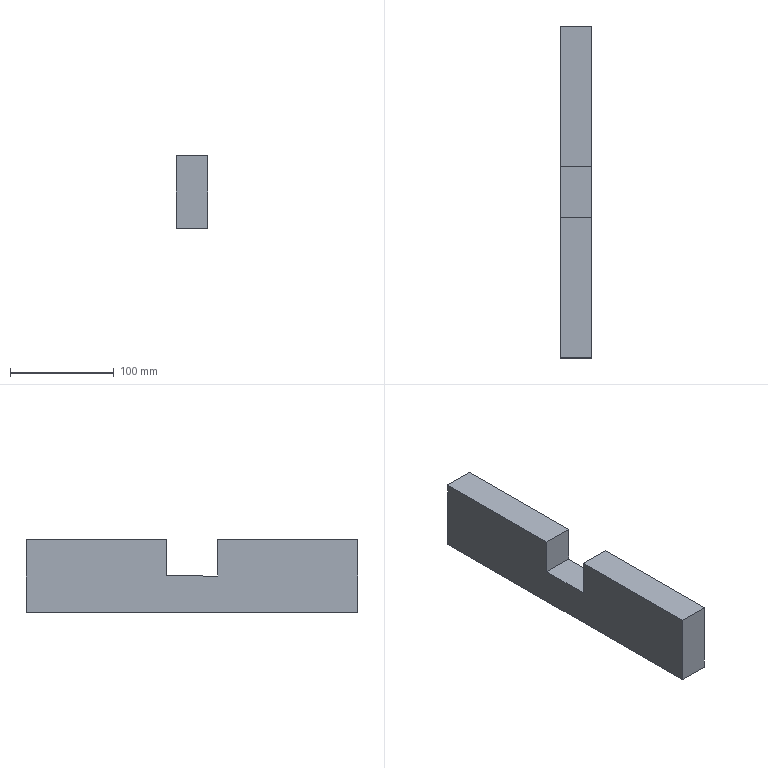Component | SolidWorks | Support5-1 | 1 solid | 10 faces | box 30 x 320 x 70 mm | volume 619500 mm3 | plane 10 | material Plain Carbon Steel
STEP:
#1=COLOUR_RGB('',0.7922,0.8196,0.9333);
#2=FILL_AREA_STYLE_COLOUR('',#1);
#3=FILL_AREA_STYLE('',(#2));
#4=SURFACE_STYLE_FILL_AREA(#3);
#5=SURFACE_SIDE_STYLE('',(#4));
#6=SURFACE_STYLE_USAGE(.BOTH.,#5);
#7=PRESENTATION_STYLE_ASSIGNMENT((#6));
#8=CARTESIAN_POINT('',(49.826,48.478,64.216));
#9=VERTEX_POINT('',#8);
#10=CARTESIAN_POINT('',(49.826,43.163,64.216));
#11=VERTEX_POINT('',#10);
#12=CARTESIAN_POINT('',(49.826,48.478,64.216));
#13=DIRECTION('',(0.,-1.,-0.));
#14=VECTOR('',#13,39.37);
#15=LINE('',#12,#14);
#16=EDGE_CURVE('',#9,#11,#15,.T.);
#17=ORIENTED_EDGE('',*,*,#16,.F.);
#18=CARTESIAN_POINT('',(48.645,48.478,64.216));
#19=VERTEX_POINT('',#18);
#20=CARTESIAN_POINT('',(48.645,48.478,64.216));
#21=DIRECTION('',(1.,0.,0.));
#22=VECTOR('',#21,39.37);
#23=LINE('',#20,#22);
#24=EDGE_CURVE('',#19,#9,#23,.T.);
#25=ORIENTED_EDGE('',*,*,#24,.F.);
#26=CARTESIAN_POINT('',(48.645,43.163,64.216));
#27=VERTEX_POINT('',#26);
#28=CARTESIAN_POINT('',(48.645,48.478,64.216));
#29=DIRECTION('',(0.,-1.,-0.));
#30=VECTOR('',#29,39.37);
#31=LINE('',#28,#30);
#32=EDGE_CURVE('',#19,#27,#31,.T.);
#33=ORIENTED_EDGE('',*,*,#32,.T.);
#34=CARTESIAN_POINT('',(48.645,43.163,64.216));
#35=DIRECTION('',(1.,0.,0.));
#36=VECTOR('',#35,39.37);
#37=LINE('',#34,#36);
#38=EDGE_CURVE('',#27,#11,#37,.T.);
#39=ORIENTED_EDGE('',*,*,#38,.T.);
#40=EDGE_LOOP('',(#17,#25,#33,#39));
#41=FACE_OUTER_BOUND('',#40,.T.);
#42=CARTESIAN_POINT('',(48.645,48.478,64.216));
#43=DIRECTION('',(0.,-0.,1.));
#44=DIRECTION('',(0.,-1.,-0.));
#45=AXIS2_PLACEMENT_3D('',#42,#43,#44);
#46=PLANE('',#45);
#47=ADVANCED_FACE('',(#41),#46,.T.);
#48=CARTESIAN_POINT('',(49.826,48.478,62.838));
#49=VERTEX_POINT('',#48);
#50=CARTESIAN_POINT('',(49.826,48.478,62.838));
#51=DIRECTION('',(0.,-0.,1.));
#52=VECTOR('',#51,39.37);
#53=LINE('',#50,#52);
#54=EDGE_CURVE('',#49,#9,#53,.T.);
#55=ORIENTED_EDGE('',*,*,#54,.F.);
#56=CARTESIAN_POINT('',(48.645,48.478,62.838));
#57=VERTEX_POINT('',#56);
#58=CARTESIAN_POINT('',(48.645,48.478,62.838));
#59=DIRECTION('',(1.,0.,0.));
#60=VECTOR('',#59,39.37);
#61=LINE('',#58,#60);
#62=EDGE_CURVE('',#57,#49,#61,.T.);
#63=ORIENTED_EDGE('',*,*,#62,.F.);
#64=CARTESIAN_POINT('',(48.645,48.478,62.838));
#65=DIRECTION('',(0.,-0.,1.));
#66=VECTOR('',#65,39.37);
#67=LINE('',#64,#66);
#68=EDGE_CURVE('',#57,#19,#67,.T.);
#69=ORIENTED_EDGE('',*,*,#68,.T.);
#70=ORIENTED_EDGE('',*,*,#24,.T.);
#71=EDGE_LOOP('',(#55,#63,#69,#70));
#72=FACE_OUTER_BOUND('',#71,.T.);
#73=CARTESIAN_POINT('',(48.645,48.478,62.838));
#74=DIRECTION('',(0.,1.,0.));
#75=DIRECTION('',(0.,-0.,1.));
#76=AXIS2_PLACEMENT_3D('',#73,#74,#75);
#77=PLANE('',#76);
#78=ADVANCED_FACE('',(#72),#77,.T.);
#79=CARTESIAN_POINT('',(49.826,50.447,62.838));
#80=VERTEX_POINT('',#79);
#81=CARTESIAN_POINT('',(49.826,50.447,62.838));
#82=DIRECTION('',(0.,-1.,-0.));
#83=VECTOR('',#82,39.37);
#84=LINE('',#81,#83);
#85=EDGE_CURVE('',#80,#49,#84,.T.);
#86=ORIENTED_EDGE('',*,*,#85,.F.);
#87=CARTESIAN_POINT('',(48.645,50.447,62.838));
#88=VERTEX_POINT('',#87);
#89=CARTESIAN_POINT('',(48.645,50.447,62.838));
#90=DIRECTION('',(1.,0.,0.));
#91=VECTOR('',#90,39.37);
#92=LINE('',#89,#91);
#93=EDGE_CURVE('',#88,#80,#92,.T.);
#94=ORIENTED_EDGE('',*,*,#93,.F.);
#95=CARTESIAN_POINT('',(48.645,50.447,62.838));
#96=DIRECTION('',(0.,-1.,-0.));
#97=VECTOR('',#96,39.37);
#98=LINE('',#95,#97);
#99=EDGE_CURVE('',#88,#57,#98,.T.);
#100=ORIENTED_EDGE('',*,*,#99,.T.);
#101=ORIENTED_EDGE('',*,*,#62,.T.);
#102=EDGE_LOOP('',(#86,#94,#100,#101));
#103=FACE_OUTER_BOUND('',#102,.T.);
#104=CARTESIAN_POINT('',(48.645,50.447,62.838));
#105=DIRECTION('',(0.,-0.,1.));
#106=DIRECTION('',(0.,-1.,-0.));
#107=AXIS2_PLACEMENT_3D('',#104,#105,#106);
#108=PLANE('',#107);
#109=ADVANCED_FACE('',(#103),#108,.T.);
#110=CARTESIAN_POINT('',(49.826,50.447,64.216));
#111=VERTEX_POINT('',#110);
#112=CARTESIAN_POINT('',(49.826,50.447,64.216));
#113=DIRECTION('',(0.,0.,-1.));
#114=VECTOR('',#113,39.37);
#115=LINE('',#112,#114);
#116=EDGE_CURVE('',#111,#80,#115,.T.);
#117=ORIENTED_EDGE('',*,*,#116,.F.);
#118=CARTESIAN_POINT('',(48.645,50.447,64.216));
#119=VERTEX_POINT('',#118);
#120=CARTESIAN_POINT('',(48.645,50.447,64.216));
#121=DIRECTION('',(1.,0.,0.));
#122=VECTOR('',#121,39.37);
#123=LINE('',#120,#122);
#124=EDGE_CURVE('',#119,#111,#123,.T.);
#125=ORIENTED_EDGE('',*,*,#124,.F.);
#126=CARTESIAN_POINT('',(48.645,50.447,64.216));
#127=DIRECTION('',(0.,0.,-1.));
#128=VECTOR('',#127,39.37);
#129=LINE('',#126,#128);
#130=EDGE_CURVE('',#119,#88,#129,.T.);
#131=ORIENTED_EDGE('',*,*,#130,.T.);
#132=ORIENTED_EDGE('',*,*,#93,.T.);
#133=EDGE_LOOP('',(#117,#125,#131,#132));
#134=FACE_OUTER_BOUND('',#133,.T.);
#135=CARTESIAN_POINT('',(48.645,50.447,64.216));
#136=DIRECTION('',(0.,-1.,-0.));
#137=DIRECTION('',(-1.,0.,0.));
#138=AXIS2_PLACEMENT_3D('',#135,#136,#137);
#139=PLANE('',#138);
#140=ADVANCED_FACE('',(#134),#139,.T.);
#141=CARTESIAN_POINT('',(49.826,55.762,64.216));
#142=VERTEX_POINT('',#141);
#143=CARTESIAN_POINT('',(49.826,55.762,64.216));
#144=DIRECTION('',(0.,-1.,-0.));
#145=VECTOR('',#144,39.37);
#146=LINE('',#143,#145);
#147=EDGE_CURVE('',#142,#111,#146,.T.);
#148=ORIENTED_EDGE('',*,*,#147,.F.);
#149=CARTESIAN_POINT('',(48.645,55.762,64.216));
#150=VERTEX_POINT('',#149);
#151=CARTESIAN_POINT('',(48.645,55.762,64.216));
#152=DIRECTION('',(1.,0.,0.));
#153=VECTOR('',#152,39.37);
#154=LINE('',#151,#153);
#155=EDGE_CURVE('',#150,#142,#154,.T.);
#156=ORIENTED_EDGE('',*,*,#155,.F.);
#157=CARTESIAN_POINT('',(48.645,55.762,64.216));
#158=DIRECTION('',(0.,-1.,-0.));
#159=VECTOR('',#158,39.37);
#160=LINE('',#157,#159);
#161=EDGE_CURVE('',#150,#119,#160,.T.);
#162=ORIENTED_EDGE('',*,*,#161,.T.);
#163=ORIENTED_EDGE('',*,*,#124,.T.);
#164=EDGE_LOOP('',(#148,#156,#162,#163));
#165=FACE_OUTER_BOUND('',#164,.T.);
#166=CARTESIAN_POINT('',(48.645,55.762,64.216));
#167=DIRECTION('',(0.,-0.,1.));
#168=DIRECTION('',(0.,-1.,-0.));
#169=AXIS2_PLACEMENT_3D('',#166,#167,#168);
#170=PLANE('',#169);
#171=ADVANCED_FACE('',(#165),#170,.T.);
#172=CARTESIAN_POINT('',(49.826,55.762,61.46));
#173=VERTEX_POINT('',#172);
#174=CARTESIAN_POINT('',(49.826,55.762,61.46));
#175=DIRECTION('',(0.,-0.,1.));
#176=VECTOR('',#175,39.37);
#177=LINE('',#174,#176);
#178=EDGE_CURVE('',#173,#142,#177,.T.);
#179=ORIENTED_EDGE('',*,*,#178,.F.);
#180=CARTESIAN_POINT('',(48.645,55.762,61.46));
#181=VERTEX_POINT('',#180);
#182=CARTESIAN_POINT('',(48.645,55.762,61.46));
#183=DIRECTION('',(1.,0.,0.));
#184=VECTOR('',#183,39.37);
#185=LINE('',#182,#184);
#186=EDGE_CURVE('',#181,#173,#185,.T.);
#187=ORIENTED_EDGE('',*,*,#186,.F.);
#188=CARTESIAN_POINT('',(48.645,55.762,61.46));
#189=DIRECTION('',(0.,-0.,1.));
#190=VECTOR('',#189,39.37);
#191=LINE('',#188,#190);
#192=EDGE_CURVE('',#181,#150,#191,.T.);
#193=ORIENTED_EDGE('',*,*,#192,.T.);
#194=ORIENTED_EDGE('',*,*,#155,.T.);
#195=EDGE_LOOP('',(#179,#187,#193,#194));
#196=FACE_OUTER_BOUND('',#195,.T.);
#197=CARTESIAN_POINT('',(48.645,55.762,61.46));
#198=DIRECTION('',(0.,1.,0.));
#199=DIRECTION('',(0.,-0.,1.));
#200=AXIS2_PLACEMENT_3D('',#197,#198,#199);
#201=PLANE('',#200);
#202=ADVANCED_FACE('',(#196),#201,.T.);
#203=CARTESIAN_POINT('',(49.826,43.163,61.46));
#204=VERTEX_POINT('',#203);
#205=CARTESIAN_POINT('',(49.826,55.762,61.46));
#206=DIRECTION('',(0.,1.,0.));
#207=VECTOR('',#206,39.37);
#208=LINE('',#205,#207);
#209=EDGE_CURVE('',#204,#173,#208,.T.);
#210=ORIENTED_EDGE('',*,*,#209,.F.);
#211=CARTESIAN_POINT('',(48.645,43.163,61.46));
#212=VERTEX_POINT('',#211);
#213=CARTESIAN_POINT('',(48.645,43.163,61.46));
#214=DIRECTION('',(1.,0.,0.));
#215=VECTOR('',#214,39.37);
#216=LINE('',#213,#215);
#217=EDGE_CURVE('',#212,#204,#216,.T.);
#218=ORIENTED_EDGE('',*,*,#217,.F.);
#219=CARTESIAN_POINT('',(48.645,55.762,61.46));
#220=DIRECTION('',(0.,1.,0.));
#221=VECTOR('',#220,39.37);
#222=LINE('',#219,#221);
#223=EDGE_CURVE('',#212,#181,#222,.T.);
#224=ORIENTED_EDGE('',*,*,#223,.T.);
#225=ORIENTED_EDGE('',*,*,#186,.T.);
#226=EDGE_LOOP('',(#210,#218,#224,#225));
#227=FACE_OUTER_BOUND('',#226,.T.);
#228=CARTESIAN_POINT('',(48.645,55.762,61.46));
#229=DIRECTION('',(0.,0.,-1.));
#230=DIRECTION('',(0.,1.,0.));
#231=AXIS2_PLACEMENT_3D('',#228,#229,#230);
#232=PLANE('',#231);
#233=ADVANCED_FACE('',(#227),#232,.T.);
#234=CARTESIAN_POINT('',(49.826,43.163,61.46));
#235=DIRECTION('',(0.,0.,-1.));
#236=VECTOR('',#235,39.37);
#237=LINE('',#234,#236);
#238=EDGE_CURVE('',#11,#204,#237,.T.);
#239=ORIENTED_EDGE('',*,*,#238,.F.);
#240=ORIENTED_EDGE('',*,*,#38,.F.);
#241=CARTESIAN_POINT('',(48.645,43.163,61.46));
#242=DIRECTION('',(0.,0.,-1.));
#243=VECTOR('',#242,39.37);
#244=LINE('',#241,#243);
#245=EDGE_CURVE('',#27,#212,#244,.T.);
#246=ORIENTED_EDGE('',*,*,#245,.T.);
#247=ORIENTED_EDGE('',*,*,#217,.T.);
#248=EDGE_LOOP('',(#239,#240,#246,#247));
#249=FACE_OUTER_BOUND('',#248,.T.);
#250=CARTESIAN_POINT('',(48.645,43.163,61.46));
#251=DIRECTION('',(0.,-1.,-0.));
#252=DIRECTION('',(-1.,0.,0.));
#253=AXIS2_PLACEMENT_3D('',#250,#251,#252);
#254=PLANE('',#253);
#255=ADVANCED_FACE('',(#249),#254,.T.);
#256=ORIENTED_EDGE('',*,*,#32,.F.);
#257=ORIENTED_EDGE('',*,*,#68,.F.);
#258=ORIENTED_EDGE('',*,*,#99,.F.);
#259=ORIENTED_EDGE('',*,*,#130,.F.);
#260=ORIENTED_EDGE('',*,*,#161,.F.);
#261=ORIENTED_EDGE('',*,*,#192,.F.);
#262=ORIENTED_EDGE('',*,*,#223,.F.);
#263=ORIENTED_EDGE('',*,*,#245,.F.);
#264=EDGE_LOOP('',(#256,#257,#258,#259,#260,#261,#262,#263));
#265=FACE_OUTER_BOUND('',#264,.T.);
#266=CARTESIAN_POINT('',(48.645,49.463,62.838));
#267=DIRECTION('',(-1.,0.,0.));
#268=DIRECTION('',(0.,1.,0.));
#269=AXIS2_PLACEMENT_3D('',#266,#267,#268);
#270=PLANE('',#269);
#271=ADVANCED_FACE('',(#265),#270,.T.);
#272=ORIENTED_EDGE('',*,*,#16,.T.);
#273=ORIENTED_EDGE('',*,*,#238,.T.);
#274=ORIENTED_EDGE('',*,*,#209,.T.);
#275=ORIENTED_EDGE('',*,*,#178,.T.);
#276=ORIENTED_EDGE('',*,*,#147,.T.);
#277=ORIENTED_EDGE('',*,*,#116,.T.);
#278=ORIENTED_EDGE('',*,*,#85,.T.);
#279=ORIENTED_EDGE('',*,*,#54,.T.);
#280=EDGE_LOOP('',(#272,#273,#274,#275,#276,#277,#278,#279));
#281=FACE_OUTER_BOUND('',#280,.T.);
#282=CARTESIAN_POINT('',(49.826,49.463,62.838));
#283=DIRECTION('',(-1.,0.,0.));
#284=DIRECTION('',(0.,1.,0.));
#285=AXIS2_PLACEMENT_3D('',#282,#283,#284);
#286=PLANE('',#285);
#287=ADVANCED_FACE('',(#281),#286,.F.);
#288=CLOSED_SHELL('',(#47,#78,#109,#140,#171,#202,#233,#255,#271,#287));
#289=MANIFOLD_SOLID_BREP('',#288);
#290=STYLED_ITEM('',(#7),#289);
#291=PRESENTATION_LAYER_ASSIGNMENT('','',(#290));
#292=(LENGTH_UNIT()NAMED_UNIT(*)SI_UNIT($,.METRE.));
#293=LENGTH_MEASURE_WITH_UNIT(LENGTH_MEASURE(0.0254),#292);
#294=DIMENSIONAL_EXPONENTS(1.,0.,0.,0.,0.,0.,0.);
#295=(CONVERSION_BASED_UNIT('',#293)LENGTH_UNIT()NAMED_UNIT(#294));
#296=UNCERTAINTY_MEASURE_WITH_UNIT(LENGTH_MEASURE(0.00001),#295,'','');
#297=(NAMED_UNIT(*)PLANE_ANGLE_UNIT()SI_UNIT($,.RADIAN.));
#298=(NAMED_UNIT(*)SI_UNIT($,.STERADIAN.)SOLID_ANGLE_UNIT());
#299=(GEOMETRIC_REPRESENTATION_CONTEXT(3)GLOBAL_UNCERTAINTY_ASSIGNED_CONTEXT((#296))GLOBAL_UNIT_ASSIGNED_CONTEXT((#295,#297,#298))REPRESENTATION_CONTEXT('',''));
#300=MECHANICAL_DESIGN_GEOMETRIC_PRESENTATION_REPRESENTATION('',(#290),#299);
#301=CARTESIAN_POINT('',(0.,0.,0.));
#302=DIRECTION('',(0.,0.,1.));
#303=DIRECTION('',(1.,0.,0.));
#304=AXIS2_PLACEMENT_3D('',#301,#302,#303);
#305=(LENGTH_UNIT()NAMED_UNIT(*)SI_UNIT($,.METRE.));
#306=LENGTH_MEASURE_WITH_UNIT(LENGTH_MEASURE(0.0254),#305);
#307=DIMENSIONAL_EXPONENTS(1.,0.,0.,0.,0.,0.,0.);
#308=(CONVERSION_BASED_UNIT('',#306)LENGTH_UNIT()NAMED_UNIT(#307));
#309=UNCERTAINTY_MEASURE_WITH_UNIT(LENGTH_MEASURE(0.00001),#308,'','');
#310=(NAMED_UNIT(*)PLANE_ANGLE_UNIT()SI_UNIT($,.RADIAN.));
#311=(NAMED_UNIT(*)SI_UNIT($,.STERADIAN.)SOLID_ANGLE_UNIT());
#312=(GEOMETRIC_REPRESENTATION_CONTEXT(3)GLOBAL_UNCERTAINTY_ASSIGNED_CONTEXT((#309))GLOBAL_UNIT_ASSIGNED_CONTEXT((#308,#310,#311))REPRESENTATION_CONTEXT('',''));
#313=ADVANCED_BREP_SHAPE_REPRESENTATION('',(#289,#304),#312);